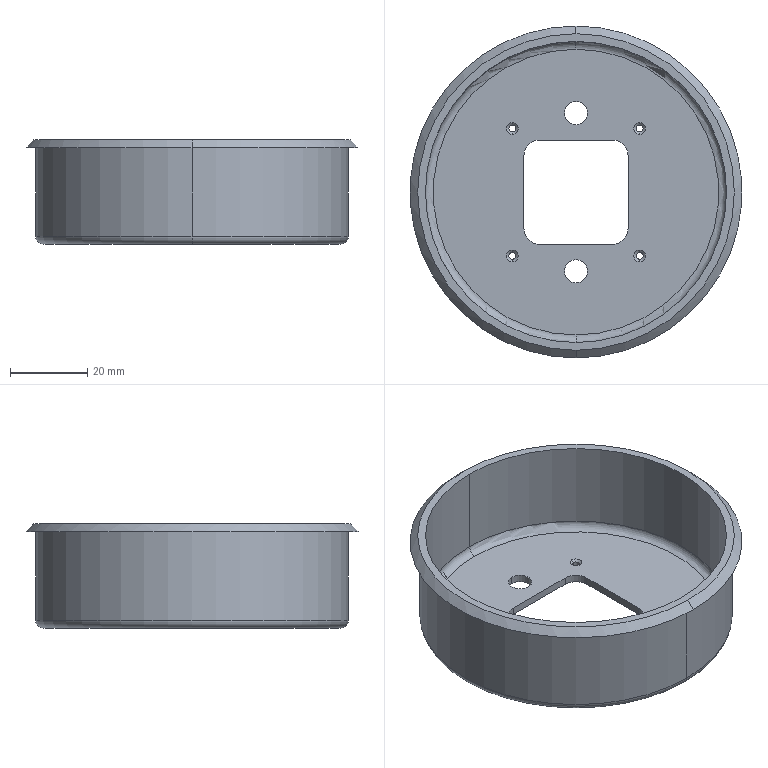Component | SolidWorks | GMotorCover2-1 | 1 solid | 42 faces | volume 18875 mm3 | cylinder 20 | cone 10 | plane 8 | torus 4 | commonest cylinder face diameters 1.778 x8 6 x4 8 x4 78 x2 81 x2